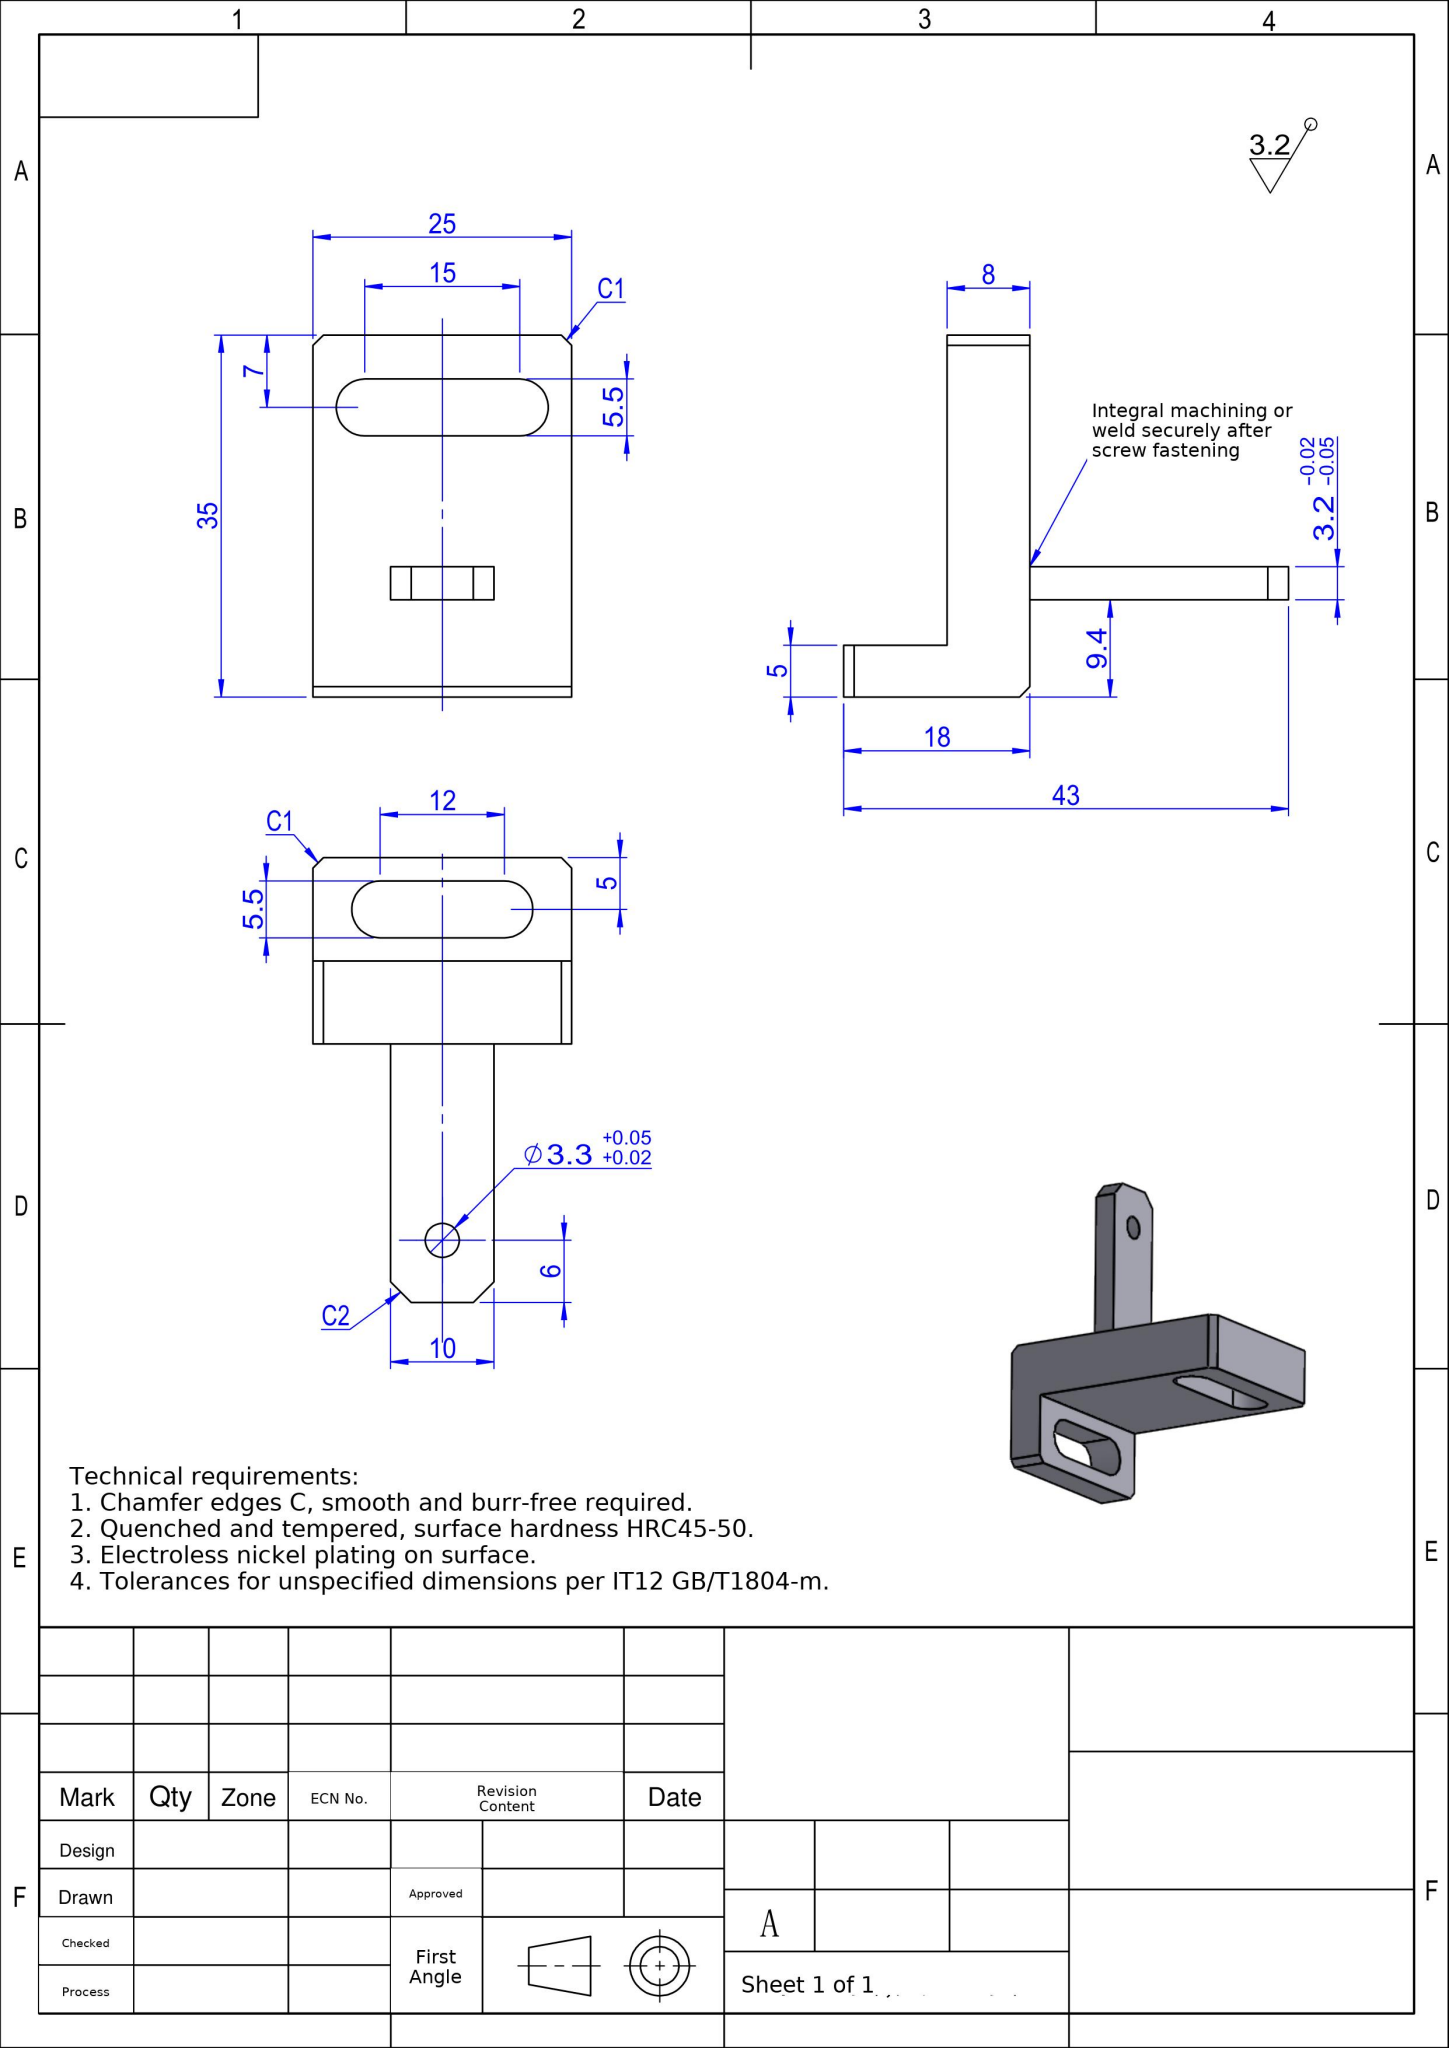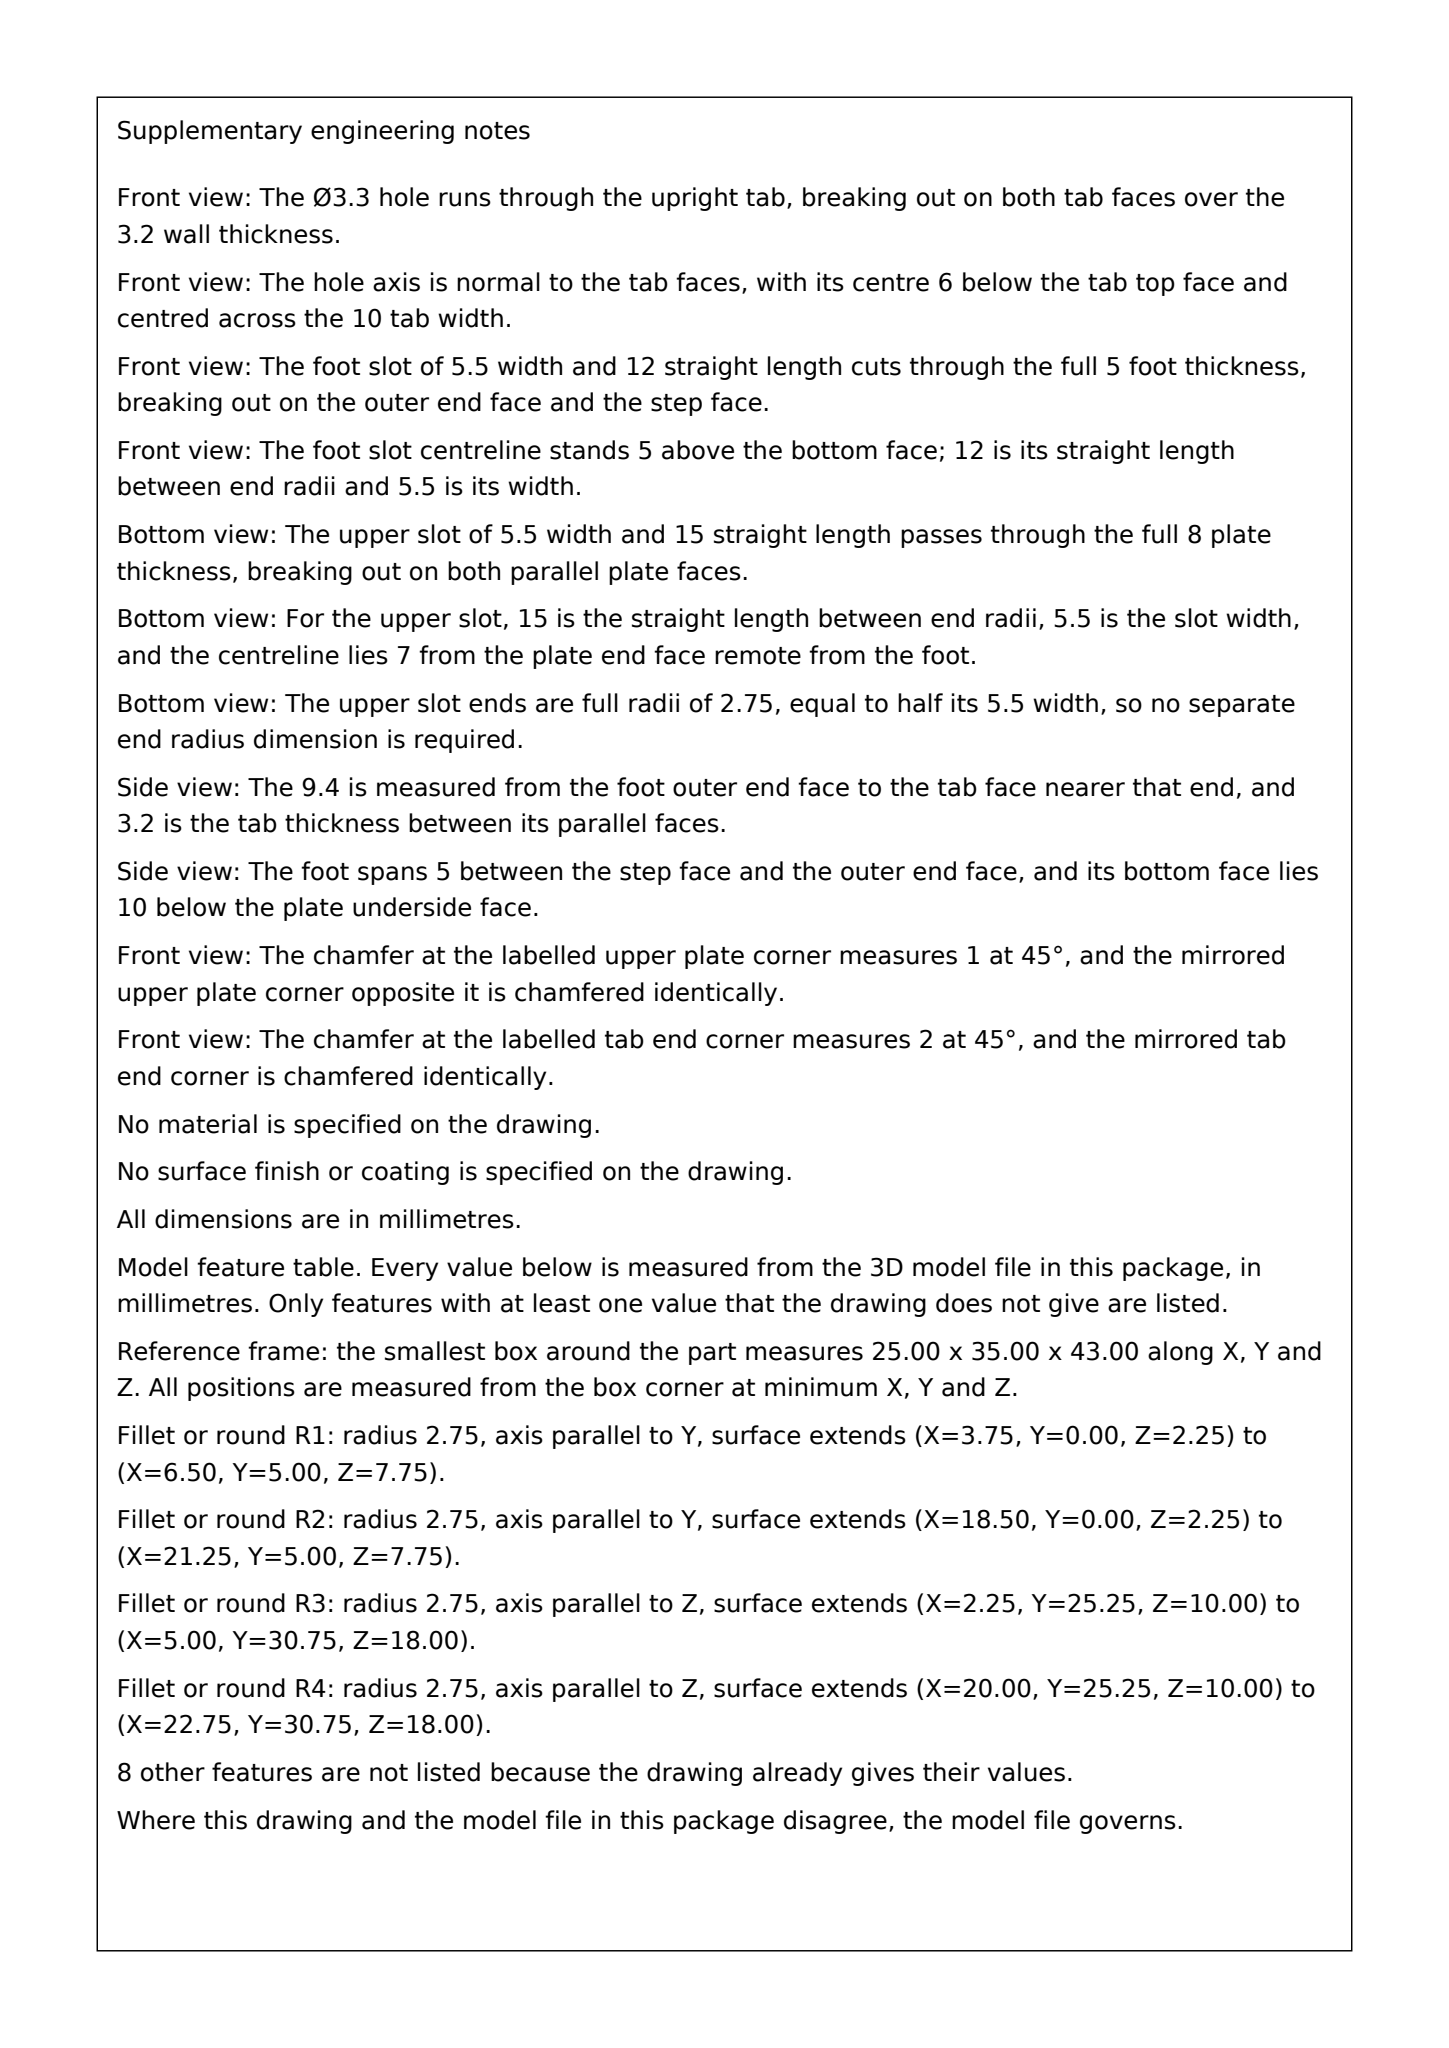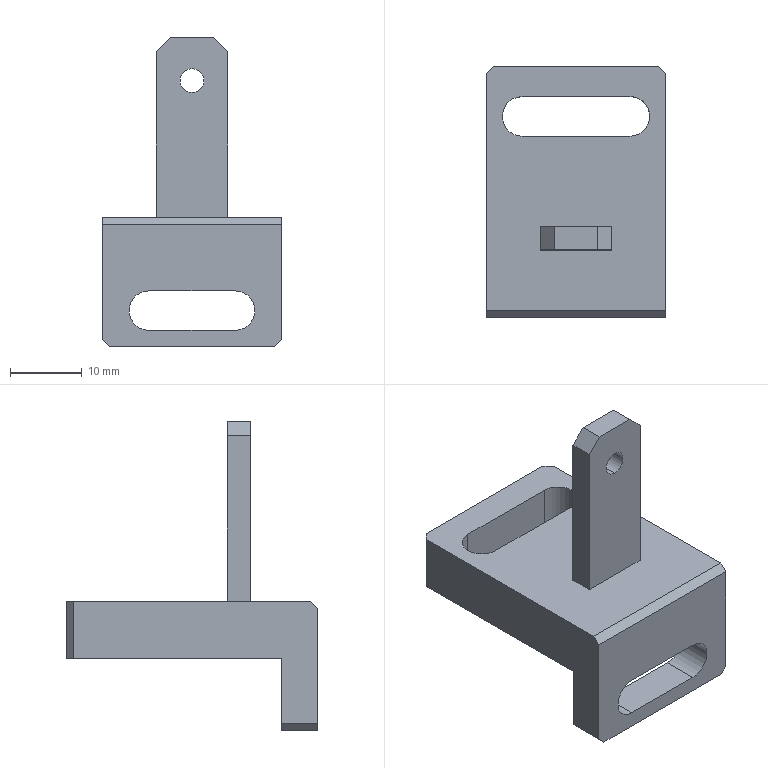Part | SolidWorks | mm | 1 solid | 31 faces | box 25 x 35 x 43 mm | volume 7685 mm3 | plane 24 | cylinder 7 | commonest cylinder face diameters 5.5 x5 3.3 x2
build123d program:
from build123d import *

# Parameters (mm, degrees)
SKETCH1_W               = 25
SKETCH1_H               = 43
BOSS_EXTRUDE1_DEPTH     = 17.5
CUT_EXTRUDE1_DEPTH      = 49.078
CUT_EXTRUDE1_DEPTH_BACK = 49.078
SKETCH2_W               = 25
SKETCH2_H               = 9.4
SKETCH2_H_2             = 22.4
SKETCH2_W_2             = 10
SKETCH2_H_3             = 30
SKETCH3_R               = 1.65
CUT_EXTRUDE2_DEPTH      = 51.07
CHAMFER1_SIZE           = 1
SKETCH6_W               = 7.5
SKETCH6_H               = 25
CUT_EXTRUDE3_DEPTH      = 52.581
CUT_EXTRUDE4_DEPTH      = 33.977
CHAMFER2_SIZE           = 2
CUT_EXTRUDE5_DEPTH      = 57.835


with BuildPart() as part:
    # Sketch1 → Boss-Extrude1 (new, symmetric)
    with BuildSketch(Plane(origin=(0, 0, 0), x_dir=(1, 0, 0), z_dir=(0, 1, 0))):
        with Locations((0, -21.5)):
            Rectangle(SKETCH1_W, SKETCH1_H)
    extrude(amount=BOSS_EXTRUDE1_DEPTH, both=True)

    # Sketch2 → Cut-Extrude1 (cut, two sides: drawn at the far end of the back side and taken through both)
    with BuildSketch(Plane(origin=(0, 0, 0), x_dir=(0, 0, -1), z_dir=(1, 0, 0)).offset(-CUT_EXTRUDE1_DEPTH_BACK)):
        with Locations((-30.5, -12.8)):
            Rectangle(SKETCH2_W, SKETCH2_H)
        with Locations((-30.5, 6.3)):
            Rectangle(SKETCH2_W, SKETCH2_H_2)
        with Locations((-5, 2.5)):
            Rectangle(SKETCH2_W_2, SKETCH2_H_3)
    extrude(amount=CUT_EXTRUDE1_DEPTH + CUT_EXTRUDE1_DEPTH_BACK, mode=Mode.SUBTRACT)

    # Sketch3 → Cut-Extrude2 (cut, through all)
    with BuildSketch(Plane(origin=(0, -4.9, 0), x_dir=(1, 0, 0), z_dir=(0, 1, 0))):
        with Locations(Location((0, -37, 0), (0, 0, 270))):
            Circle(SKETCH3_R)
    extrude(amount=-CUT_EXTRUDE2_DEPTH, mode=Mode.SUBTRACT)

    # Chamfer1
    chamfer1_edges = [part.edges().sort_by_distance(p)[0] for p in [
        (0, -17.5, 18),
        (12.5, 17.5, 14),
        (-12.5, 17.5, 14),
        (12.5, -15, 0),
        (-12.5, -15, 0),
    ]]
    chamfer(chamfer1_edges, length=CHAMFER1_SIZE)

    # Sketch6 → Cut-Extrude3 (cut, through all)
    with BuildSketch(Plane.XZ.offset(8.1)):
        with Locations((-8.75, 30.5)):
            Rectangle(SKETCH6_W, SKETCH6_H)
        with Locations((8.75, 30.5)):
            Rectangle(SKETCH6_W, SKETCH6_H)
    extrude(amount=-CUT_EXTRUDE3_DEPTH, mode=Mode.SUBTRACT)

    # Sketch7 → Cut-Extrude4 (cut, through all)
    with BuildSketch(Plane.XY.offset(18)):
        with BuildLine():
            Line((-7.5, 13.25), (7.5, 13.25))
            ThreePointArc((7.5, 13.25), (10.25, 10.5), (7.5, 7.75))
            Line((7.5, 7.75), (-7.5, 7.75))
            ThreePointArc((-7.5, 7.75), (-10.25, 10.5), (-7.5, 13.25))
        make_face()
    extrude(amount=-CUT_EXTRUDE4_DEPTH, mode=Mode.SUBTRACT)

    # Chamfer2
    chamfer2_edges = [part.edges().sort_by_distance(p)[0] for p in [
        (5, -6.5, 43),
        (-5, -6.5, 43),
    ]]
    chamfer(chamfer2_edges, length=CHAMFER2_SIZE)

    # Sketch8 → Cut-Extrude5 (cut, through all)
    with BuildSketch(Plane.XZ.offset(17.5)):
        with BuildLine():
            Line((-6, 7.75), (6, 7.75))
            ThreePointArc((6, 7.75), (8.75, 5), (6, 2.25))
            Line((6, 2.25), (-6, 2.25))
            ThreePointArc((-6, 2.25), (-8.75, 5), (-6, 7.75))
        make_face()
    extrude(amount=-CUT_EXTRUDE5_DEPTH, mode=Mode.SUBTRACT)


solid = part.part